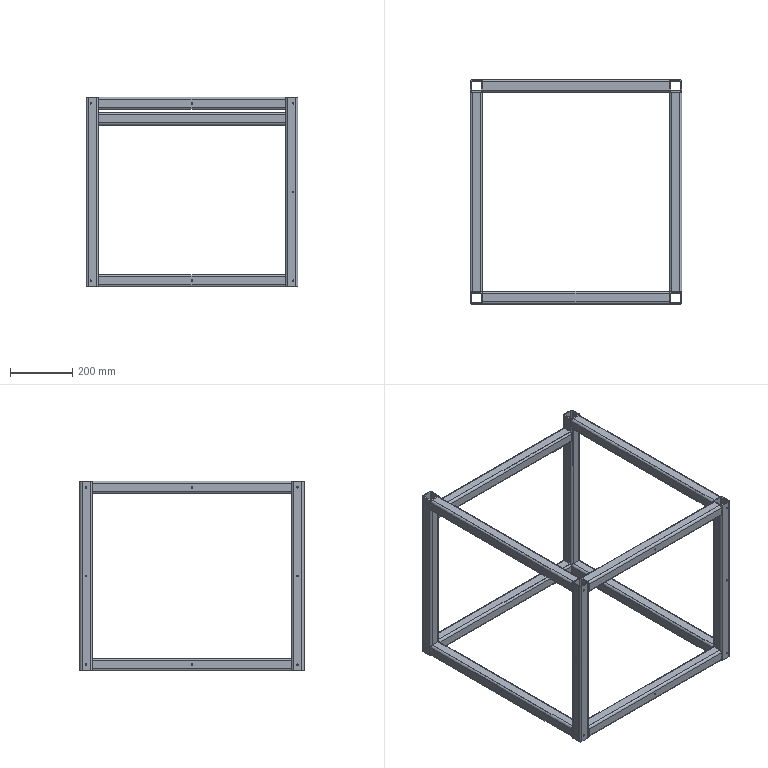Component | SolidWorks | 01-01FrameBody-1_01FrameBody-2 | 12 solids | 280 faces | volume 4005887 mm3 | cylinder 160 | plane 120 | commonest cylinder face diameters 5 x60 14 x48 6 x48 3.3 x4 | material 4040 Square Tube